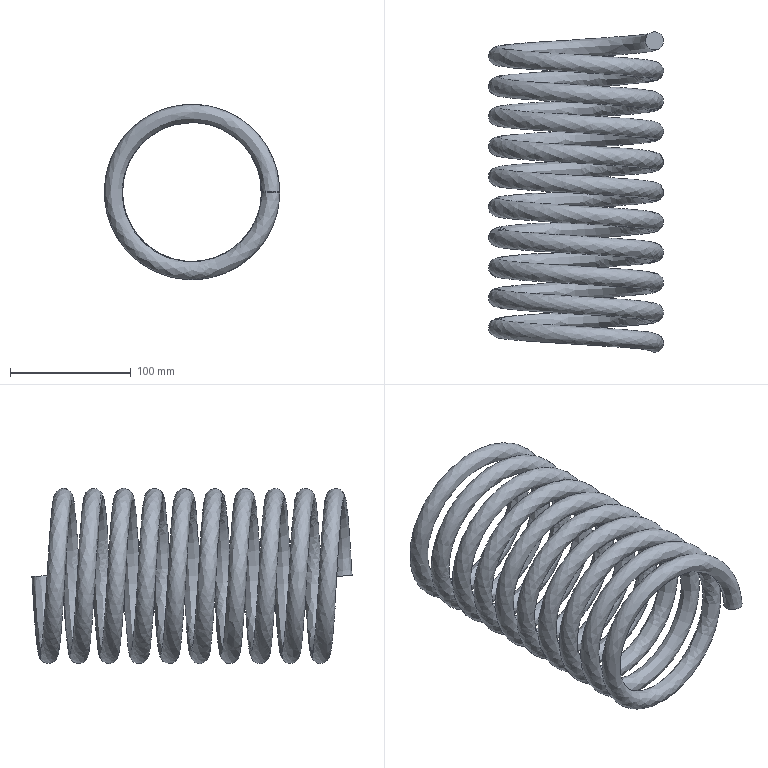Component | NX | SPRING | 1 solid | 3 faces | volume 722919 mm3 | plane 2 | spline 1